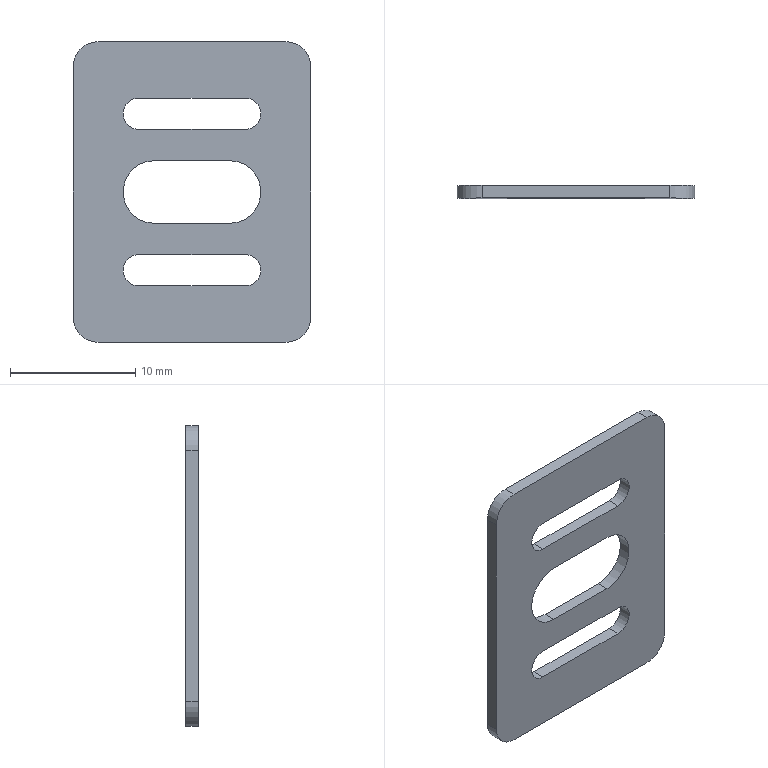Component | NX | SHIM_PLATE | 1 solid | 22 faces | volume 351 mm3 | plane 12 | cylinder 10 | commonest cylinder face diameters 2.5 x4 4 x4 5 x2